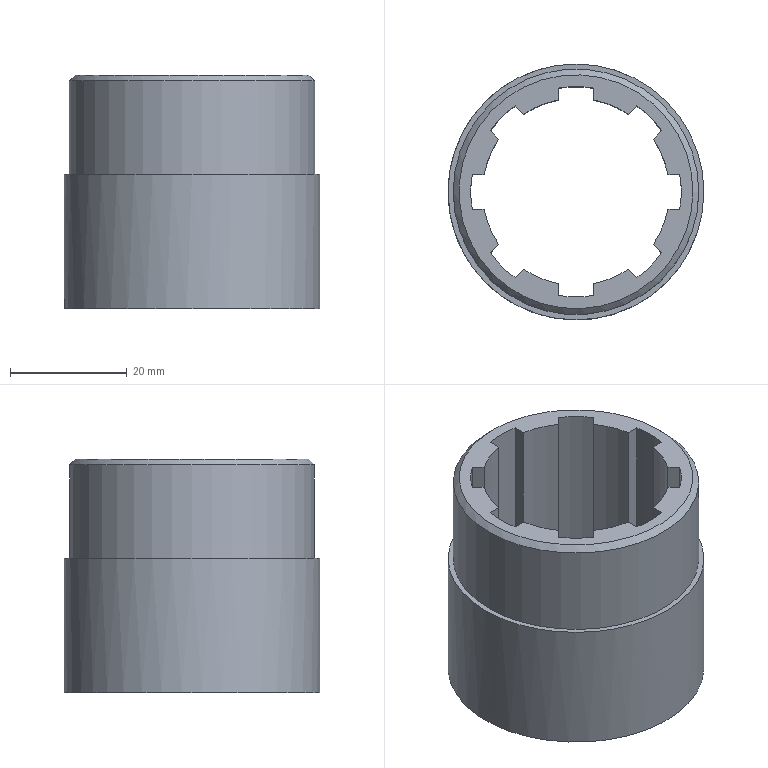Component | NX | ZYC20 | 1 solid | 38 faces | volume 22033 mm3 | plane 19 | cylinder 18 | cone 1 | commonest cylinder face diameters 32 x8 36 x8 43.75 x1 42 x1